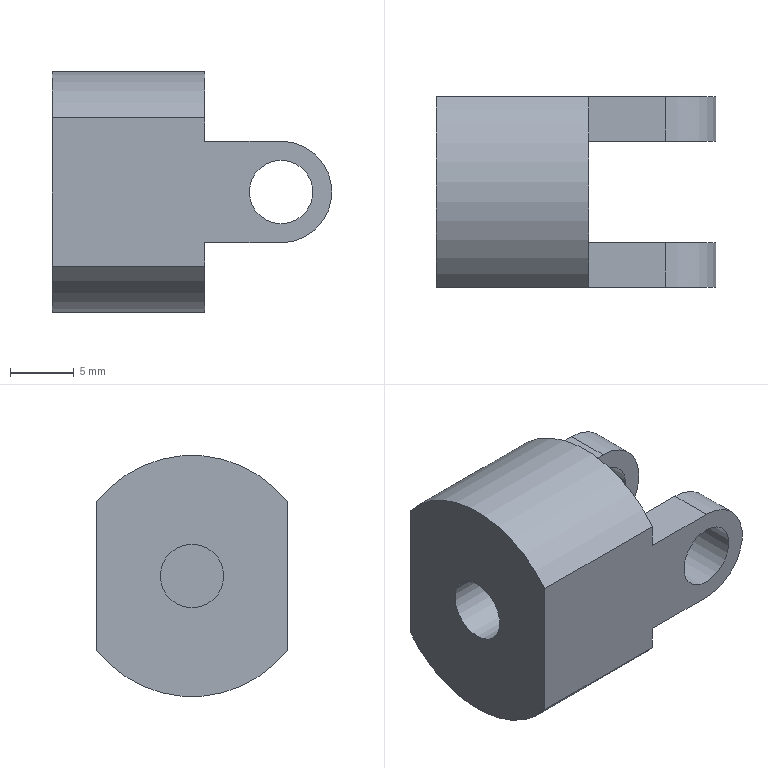Component | NX | CONNECTING_BLOCK | 1 solid | 18 faces | volume 3238 mm3 | plane 11 | cylinder 7 | commonest cylinder face diameters 5 x3 19 x2 8 x2